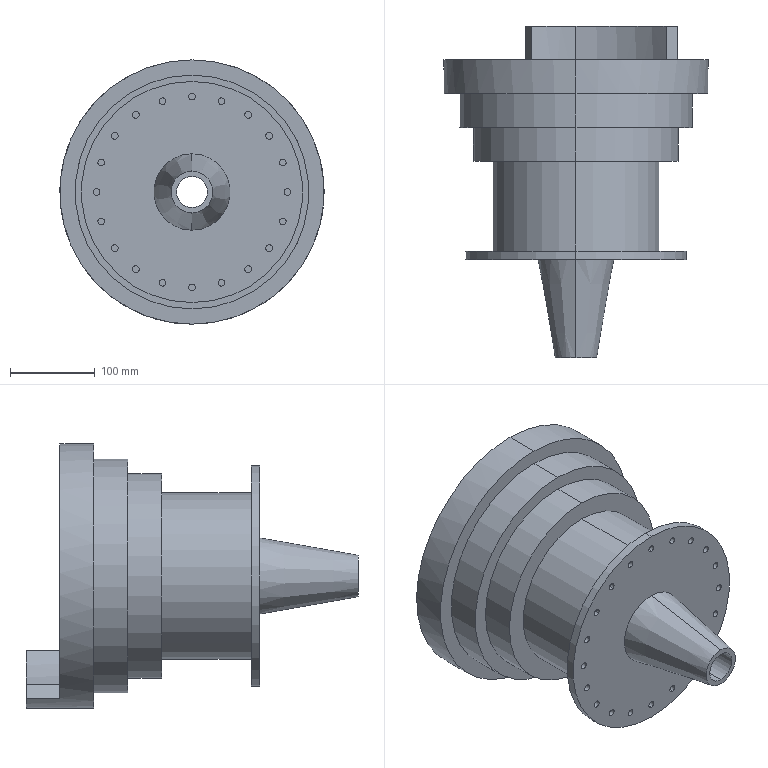Component | SolidWorks | Part24-1 | 2 solids | 67 faces | volume 8882136 mm3 | cylinder 54 | plane 11 | cone 2 | commonest cylinder face diameters 8 x40 276.036 x2 312.029 x2 261.082 x2 36.619 x2 242.018 x2 276 x2 196.008 x2